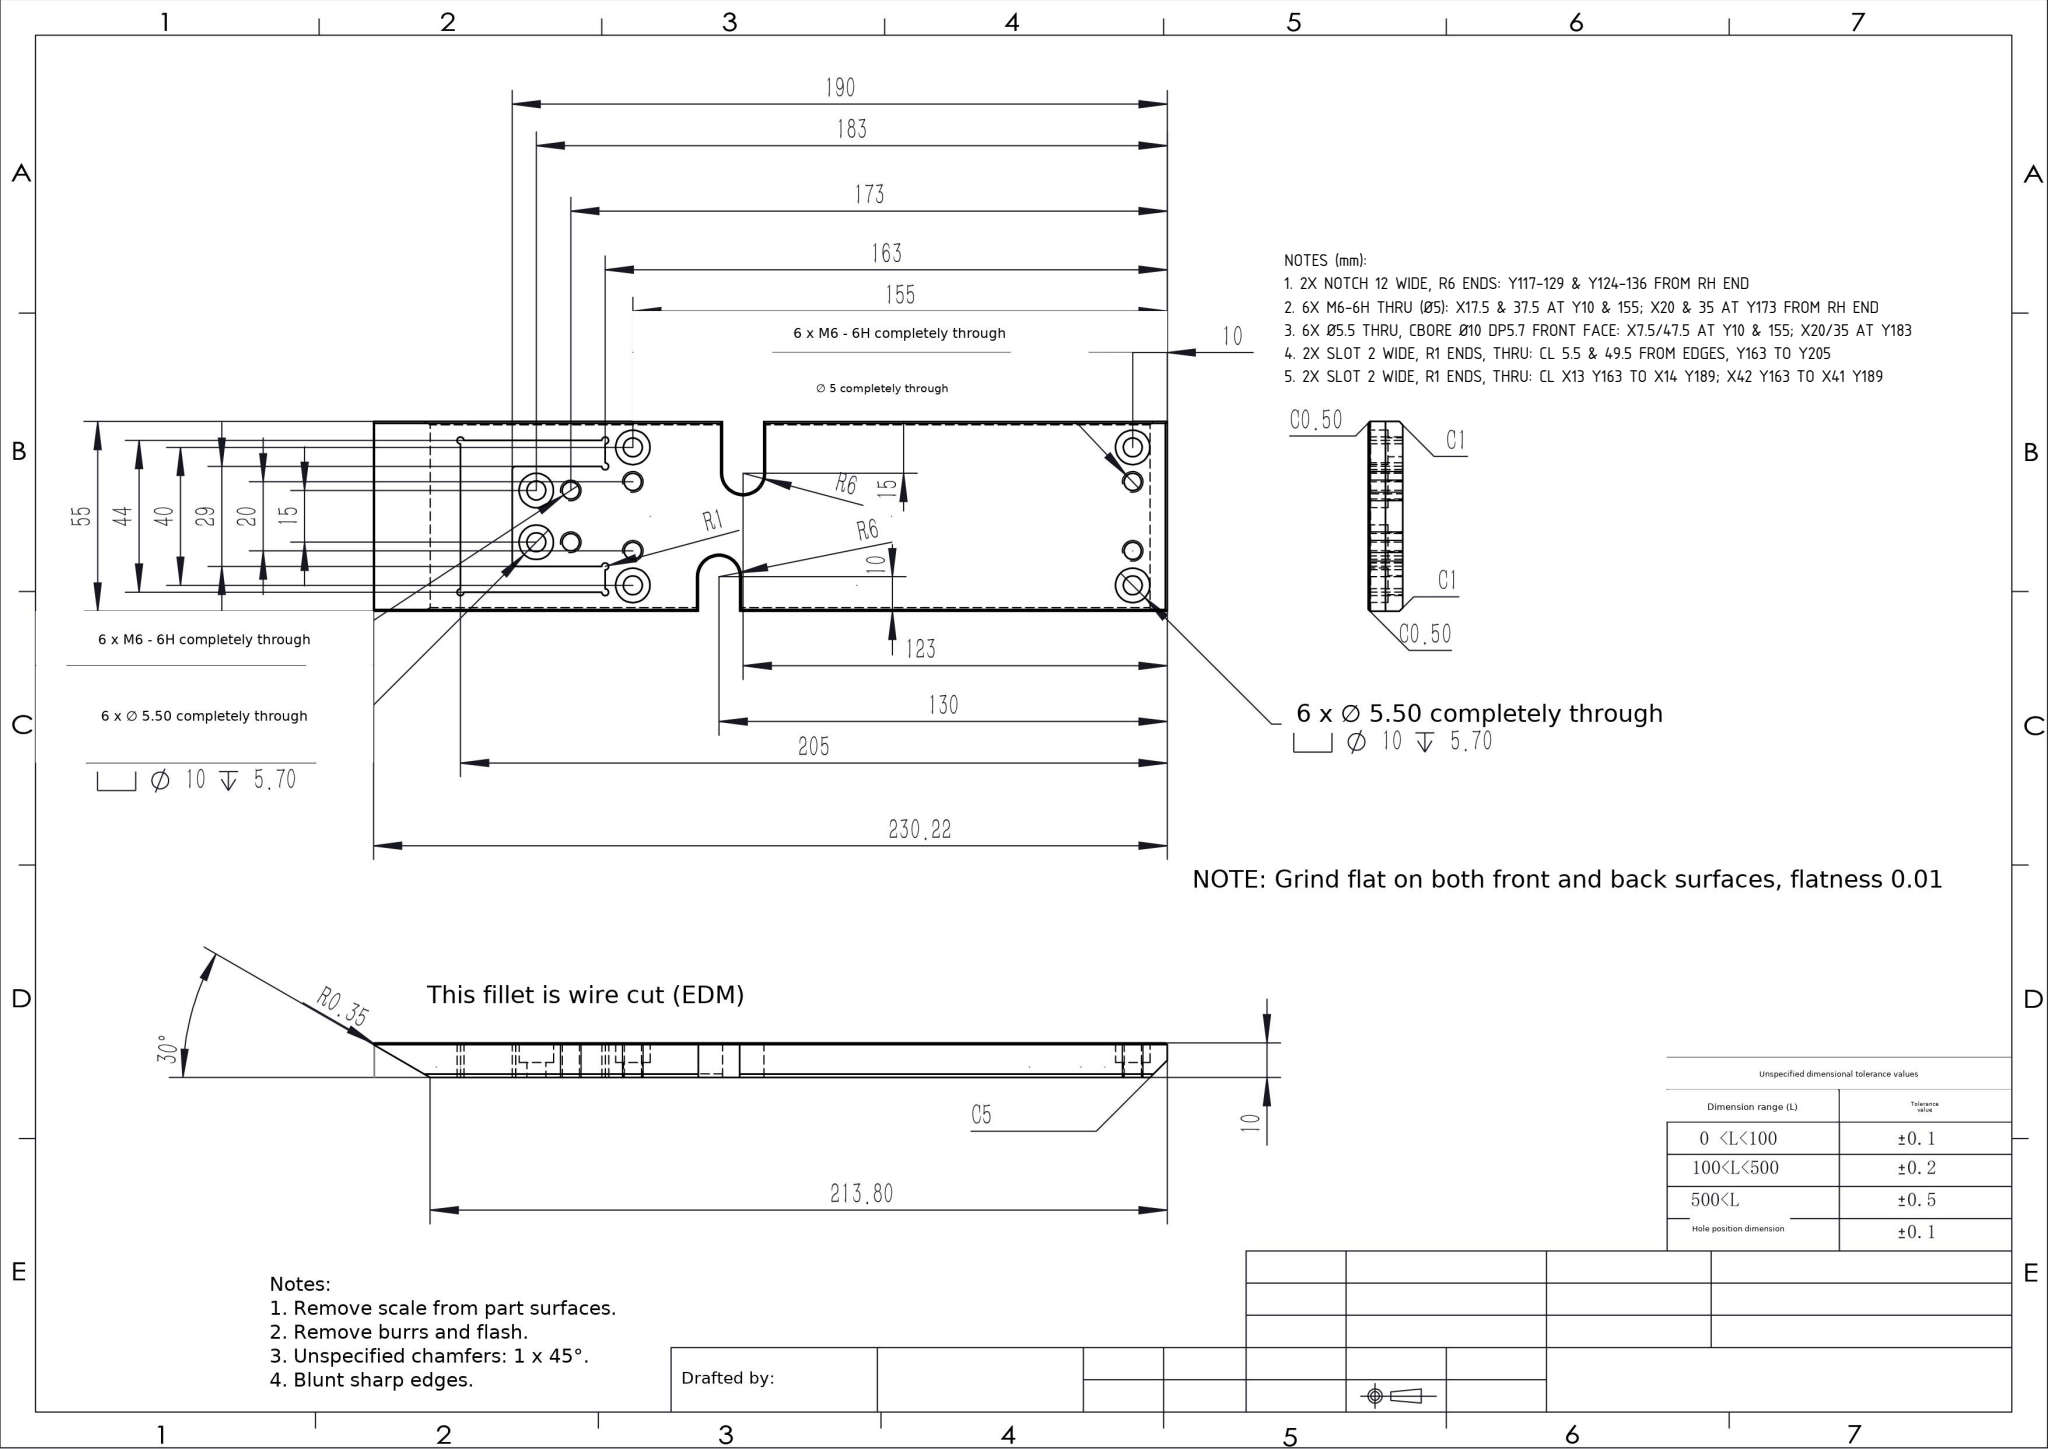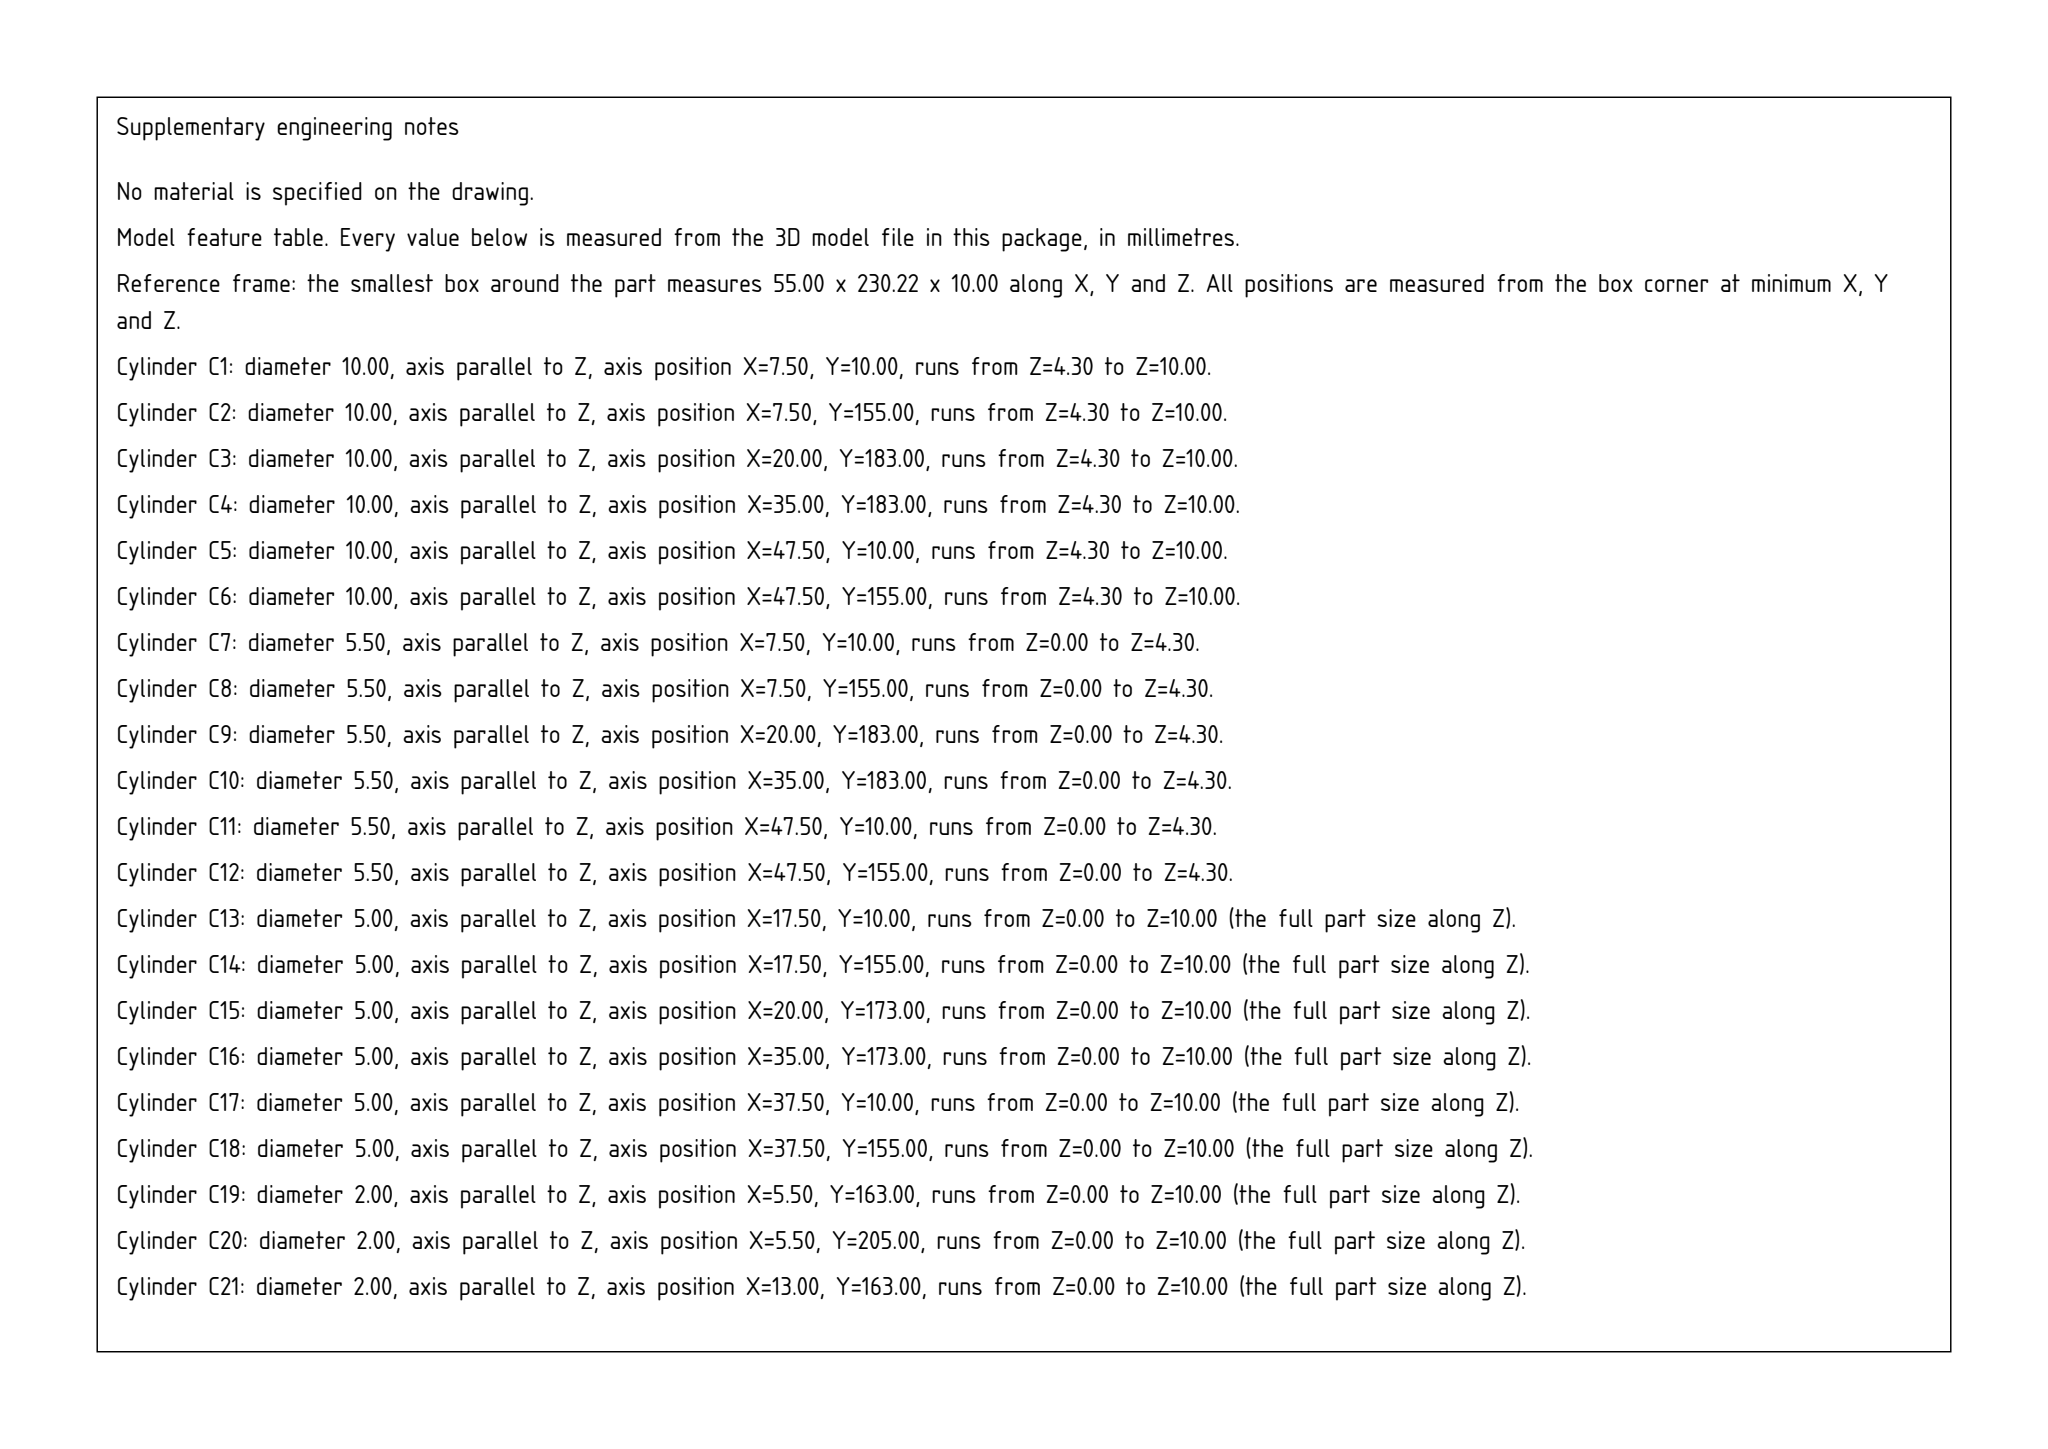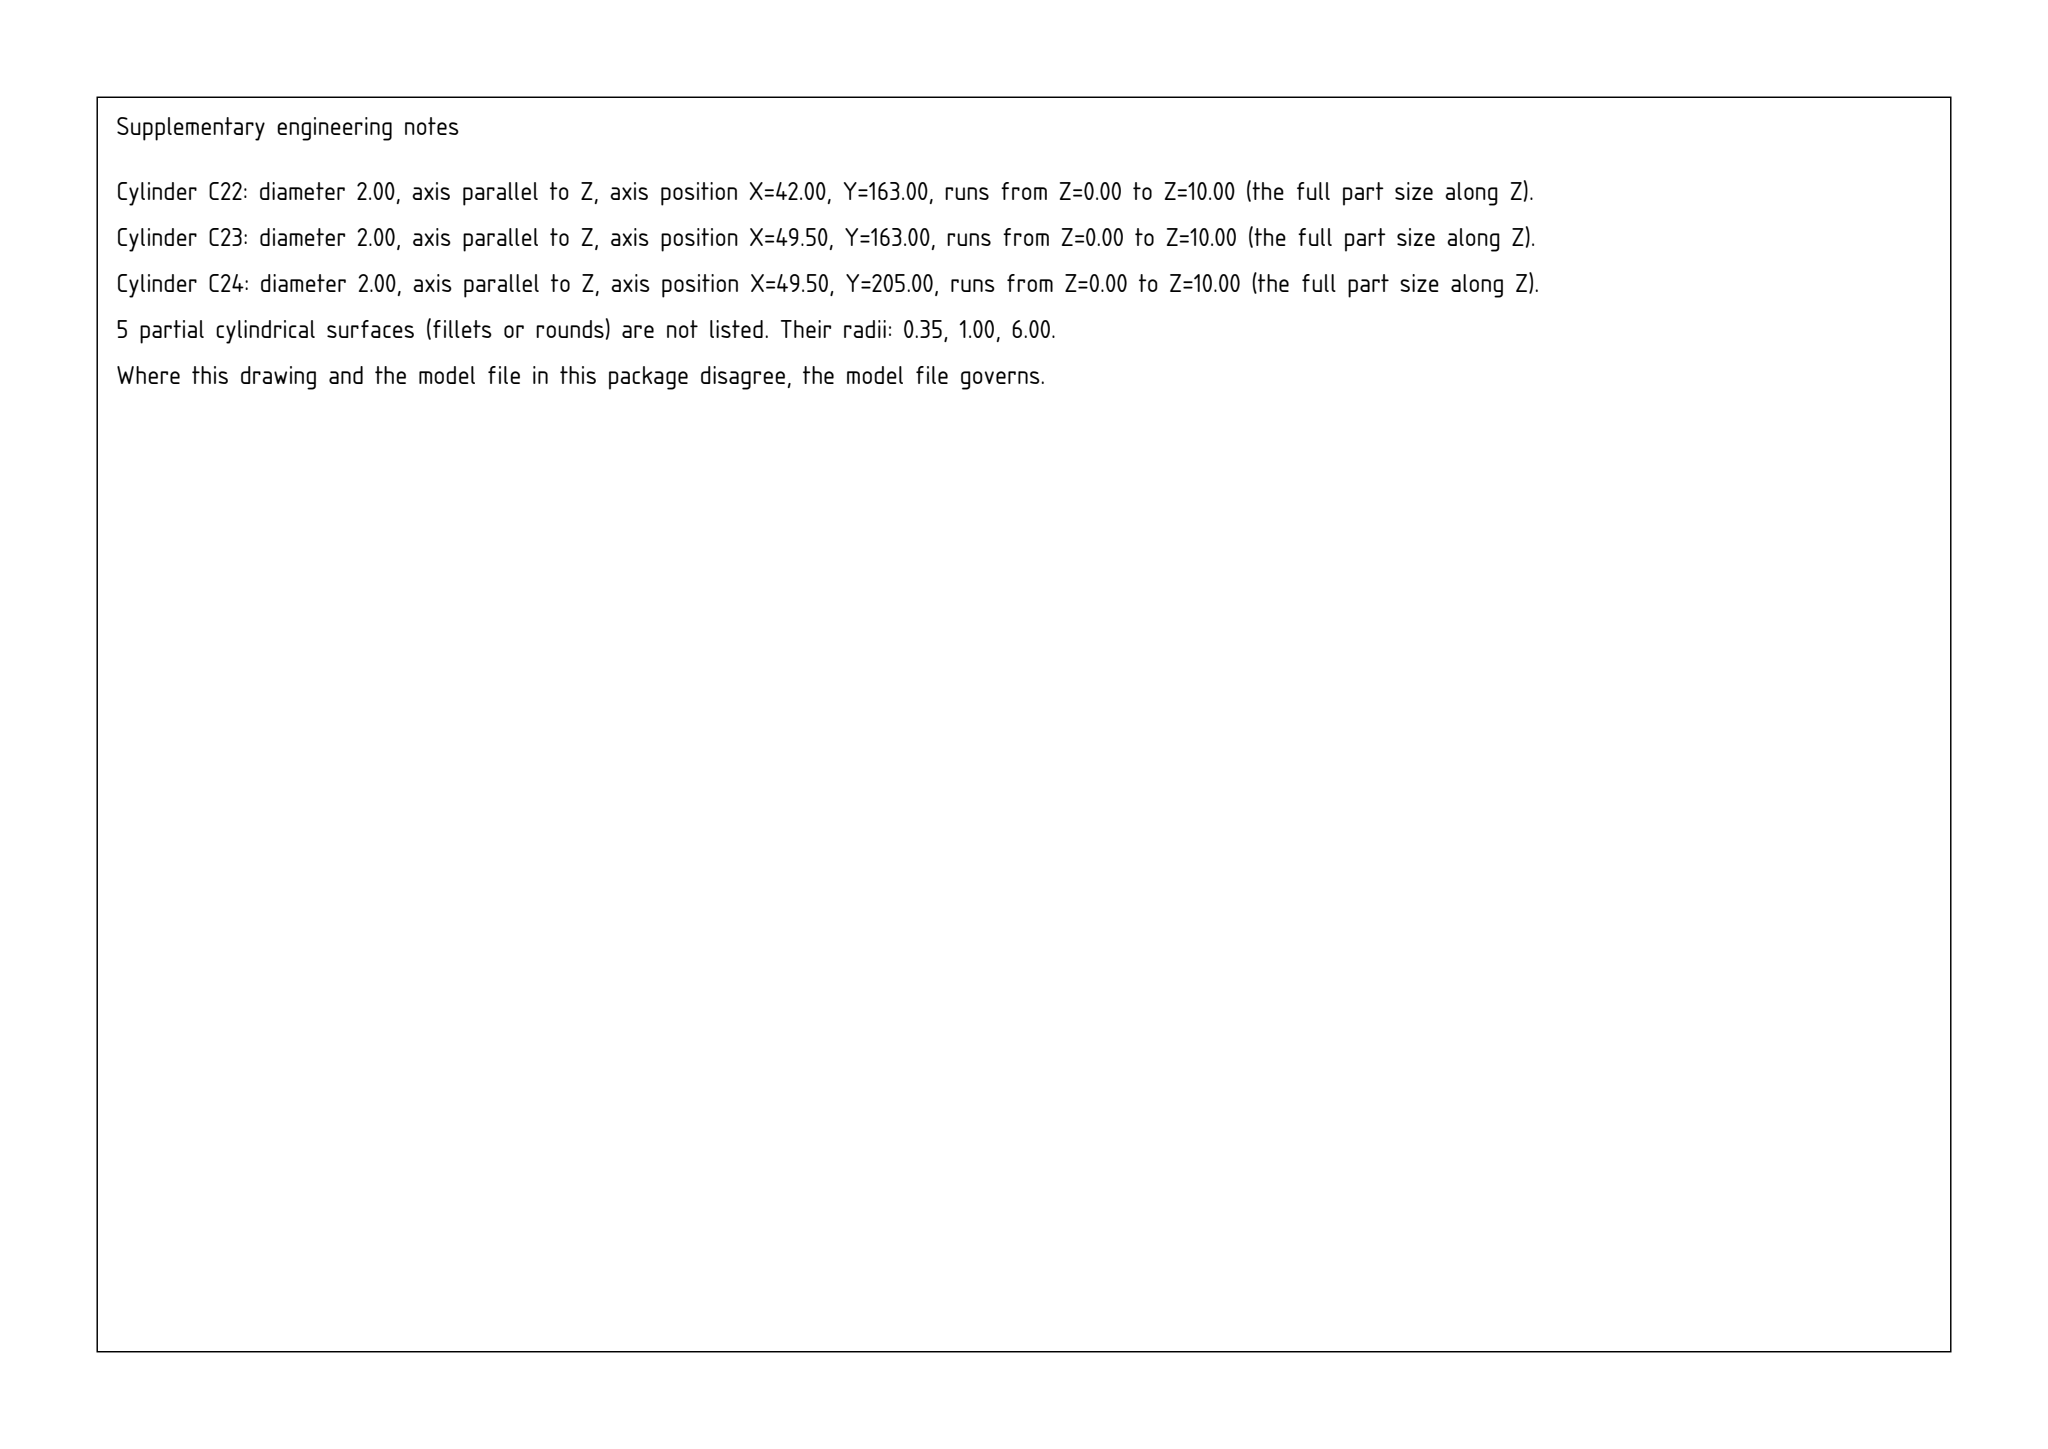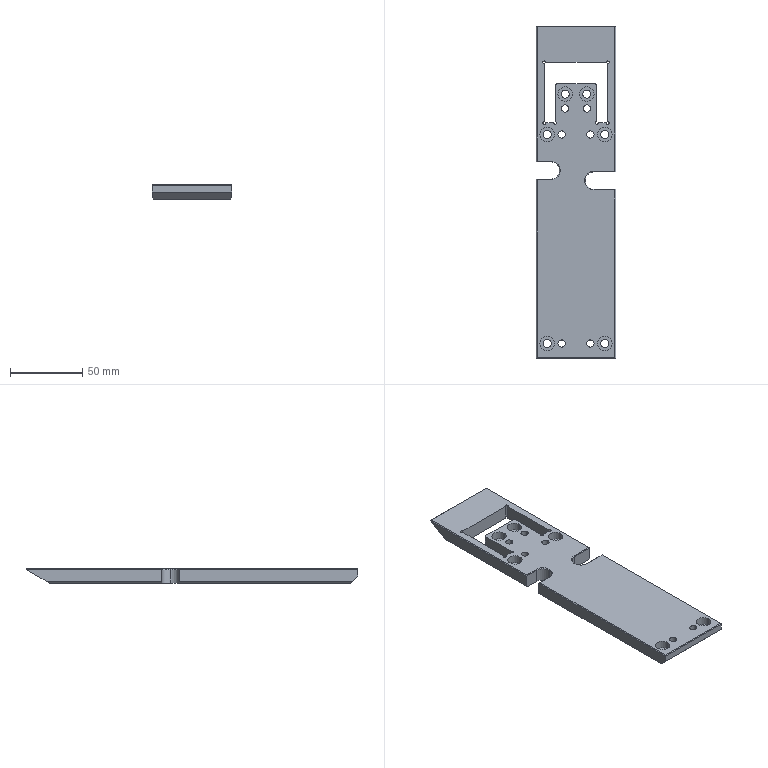Part | SolidWorks | mm | 1 solid | 95 faces | box 55 x 230.22 x 10 mm | volume 101978 mm3 | cylinder 52 | plane 40 | cone 3 | commonest cylinder face diameters 5 x12 10 x12 5.5 x12 2 x11 12 x3 0.7 x2
Drawing notes:
2X NOTCH 12 WIDE, R6 ENDS: Y117-129 & Y124-136 FROM RH END | from the solid: Ø12 cyls at y=123 (x=40) & y=130 (x=10); y-planes 117,129,124,136
6X M6-6H THRU (Ø5): X17.5 & 37.5 AT Y10 & 155; X20 & 35 AT Y173 FROM RH END | from the solid: Ø5 thru len 10 at x17.5/37.5 y=10 & 155; x20/35 y=173
6X Ø5.5 THRU, CBORE Ø10 DP5.7 FRONT FACE: X7.5/47.5 AT Y10 & 155; X20/35 AT Y183 | from the solid: Ø5.5 len 4.3 + Ø10 dp 5.7 from z=10 face, floors at z-plane 4.3
2X SLOT 2 WIDE, R1 ENDS, THRU: CL 5.5 & 49.5 FROM EDGES, Y163 TO Y205 | from the solid: Ø2 cyls len 10 at (5.5,163),(5.5,205),(49.5,163),(49.5,205)
2X SLOT 2 WIDE, R1 ENDS, THRU: CL X13 Y163 TO X14 Y189; X42 Y163 TO X41 Y189 | from the solid: Ø2 cyls len 10 at (13,163),(14,189) and mirrored (42,163),(41,189)
build123d program:
from build123d import *

# Parameters (mm, degrees)
SKETCH1_W                                            = 55
SKETCH1_H                                            = 230
BOSS_EXTRUDE1_DEPTH                                  = 10
CHAMFER7_SIZE                                        = 1
CHAMFER8_SIZE                                        = 5
SKETCH33_W                                           = 44
SKETCH33_H                                           = 42
CUT_EXTRUDE7_DEPTH                                   = 119.664
SKETCH35_W                                           = 29
SKETCH35_H                                           = 27
BOSS_EXTRUDE2_DEPTH                                  = 10
CHAMFER9_SIZE                                        = 16.2
CHAMFER9_SIZE2                                       = 9.353
BOSS_EXTRUDE3_DEPTH                                  = 55
HOLE_SIZE_ACCORDING_TO_THE_TYPE_OF_HEXAG_D           = 5.5
HOLE_SIZE_ACCORDING_TO_THE_TYPE_OF_HEXAG_CBORE_D     = 10
HOLE_SIZE_ACCORDING_TO_THE_TYPE_OF_HEXAG_CBORE_DEPTH = 5.7
M6_TAPPED_HOLE1_D                                    = 5
CUT_EXTRUDE8_DEPTH                                   = 119.874
CHAMFER10_SIZE                                       = 0.5
SKETCH38_R                                           = 1
CUT_EXTRUDE9_DEPTH                                   = 119.874
FILLET1_R                                            = 1


with BuildPart() as part:
    # Sketch1 → Boss-Extrude1 (new body)
    with BuildSketch(Plane.XY):
        Rectangle(SKETCH1_W, SKETCH1_H)
    extrude(amount=BOSS_EXTRUDE1_DEPTH)

    # Chamfer7
    chamfer7_edges = [part.edges().sort_by_distance(p)[0] for p in [
        (-27.5, 0, 0),
        (27.5, 0, 0),
    ]]
    chamfer(chamfer7_edges, length=CHAMFER7_SIZE)

    # Chamfer8
    chamfer8_edges = [part.edges().sort_by_distance(p)[0] for p in [
        (0, -115, 0),
    ]]
    chamfer(chamfer8_edges, length=CHAMFER8_SIZE)

    # Sketch33 → Cut-Extrude7 (cut, through all)
    with BuildSketch(Plane.XY.offset(10)):
        with Locations((0, 69)):
            Rectangle(SKETCH33_W, SKETCH33_H)
    extrude(amount=-CUT_EXTRUDE7_DEPTH, mode=Mode.SUBTRACT)

    # Sketch35 → Boss-Extrude2 (add)
    with BuildSketch(Plane.XY.offset(10)):
        with Locations((0, 61.5)):
            Rectangle(SKETCH35_W, SKETCH35_H)
    extrude(amount=-BOSS_EXTRUDE2_DEPTH)

    # Chamfer9
    chamfer9_edges = [part.edges().sort_by_distance(p)[0] for p in [
        (0, 115, 0),
    ]]
    chamfer9_side = [part.faces().sort_by_distance(p)[0] for p in [
        (0, -4.562, 0),
    ]]
    chamfer(chamfer9_edges, length=CHAMFER9_SIZE, length2=CHAMFER9_SIZE2, reference=chamfer9_side[0])

    # Sketch36 → Boss-Extrude3 (add)
    with BuildSketch(Plane(origin=(27.5, 0, 0), x_dir=(0, 0, -1), z_dir=(1, 0, 0))):
        with BuildLine():
            Line((-10, 115), (-9.353, 115))
            ThreePointArc((-9.353, 115), (-9.677, 115.216), (-10, 115))
        make_face()
    extrude(amount=-BOSS_EXTRUDE3_DEPTH)

    # Hole size according to the type of hexag (through all)
    with Locations(Plane.XY.offset(10)):
        with Locations((20, -105), (-20, -105), (-20, 40), (20, 40), (-7.5, 68), (7.5, 68)):
            CounterBoreHole(HOLE_SIZE_ACCORDING_TO_THE_TYPE_OF_HEXAG_D / 2, HOLE_SIZE_ACCORDING_TO_THE_TYPE_OF_HEXAG_CBORE_D / 2, HOLE_SIZE_ACCORDING_TO_THE_TYPE_OF_HEXAG_CBORE_DEPTH)

    # M6 Tapped Hole1 (through all)
    with Locations(Plane.XY.offset(10)):
        with Locations((-10, -105), (10, -105), (10, 40), (-10, 40), (-7.5, 58), (7.5, 58)):
            Hole(M6_TAPPED_HOLE1_D / 2)

    # Sketch37 → Cut-Extrude8 (cut, through all)
    with BuildSketch(Plane.XY.offset(10)):
        with BuildLine():
            Line((-47.5, 21), (-17.5, 21))
            ThreePointArc((-17.5, 21), (-11.5, 15), (-17.5, 9))
            Line((-17.5, 9), (-47.5, 9))
            ThreePointArc((-47.5, 9), (-53.5, 15), (-47.5, 21))
        make_face()
        with BuildLine():
            Line((42.5, 2), (12.5, 2))
            ThreePointArc((12.5, 2), (6.5, 8), (12.5, 14))
            Line((12.5, 14), (42.5, 14))
            ThreePointArc((42.5, 14), (48.5, 8), (42.5, 2))
        make_face()
    extrude(amount=-CUT_EXTRUDE8_DEPTH, mode=Mode.SUBTRACT)

    # Chamfer10
    chamfer10_edges = [part.edges().sort_by_distance(p)[0] for p in [
        (-27.5, 68, 10),
        (0, -115, 10),
        (-27.5, -53, 10),
        (-22.5, 21, 10),
        (-22.5, 9, 10),
        (-11.5, 15, 10),
        (27.5, 64.5, 10),
        (20, 2, 10),
        (20, 14, 10),
        (6.5, 8, 10),
        (27.5, -56.5, 10),
    ]]
    chamfer(chamfer10_edges, length=CHAMFER10_SIZE)

    # Sketch38 → Cut-Extrude9 (cut, through all)
    with BuildSketch(Plane.XY.offset(10)):
        with Locations((22, 48)):
            Circle(SKETCH38_R)
        with Locations((14.5, 48)):
            Circle(SKETCH38_R)
        with Locations((-14.5, 48)):
            Circle(SKETCH38_R)
        with Locations((-22, 48)):
            Circle(SKETCH38_R)
        with Locations((-22, 90)):
            Circle(SKETCH38_R)
        with Locations((22, 90)):
            Circle(SKETCH38_R)
    extrude(amount=-CUT_EXTRUDE9_DEPTH, mode=Mode.SUBTRACT)

    # Fillet1
    fillet1_edges = [part.edges().sort_by_distance(p)[0] for p in [
        (14.5, 75, 5),
        (-14.5, 75, 5),
    ]]
    fillet(fillet1_edges, radius=FILLET1_R)


solid = part.part